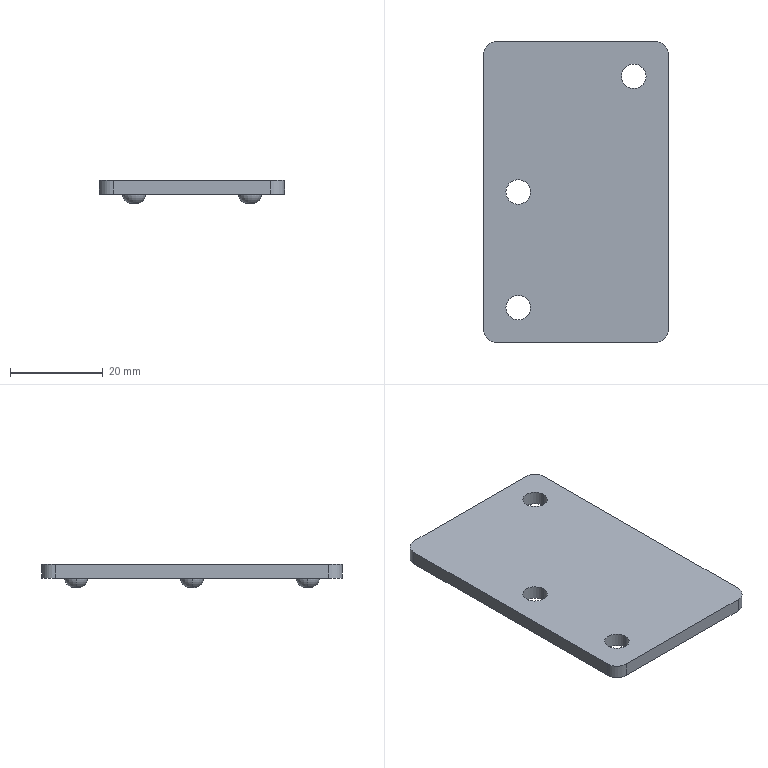Component | SolidWorks | ConnectingPlate-1 | 1 solid | 25 faces | box 40 x 65 x 5 mm | volume 7663 mm3 | cylinder 10 | plane 9 | torus 6 | commonest cylinder face diameters 5.3 x6 6 x4 | material Plain Carbon Steel
STEP:
#1=COLOUR_RGB('',0.7922,0.8196,0.9333);
#2=FILL_AREA_STYLE_COLOUR('',#1);
#3=FILL_AREA_STYLE('',(#2));
#4=SURFACE_STYLE_FILL_AREA(#3);
#5=SURFACE_SIDE_STYLE('',(#4));
#6=SURFACE_STYLE_USAGE(.BOTH.,#5);
#7=PRESENTATION_STYLE_ASSIGNMENT((#6));
#8=CARTESIAN_POINT('',(-206.949,336.302,264.226));
#9=VERTEX_POINT('',#8);
#10=CARTESIAN_POINT('',(-207.146,336.302,264.226));
#11=VERTEX_POINT('',#10);
#12=CARTESIAN_POINT('',(-207.047,336.302,264.226));
#13=DIRECTION('',(-0.,-0.,-1.));
#14=DIRECTION('',(1.,0.,-0.));
#15=AXIS2_PLACEMENT_3D('',#12,#13,#14);
#16=CIRCLE('',#15,0.09843);
#17=EDGE_CURVE('',#9,#11,#16,.T.);
#18=ORIENTED_EDGE('',*,*,#17,.T.);
#19=CARTESIAN_POINT('',(-207.067,336.302,264.147));
#20=VERTEX_POINT('',#19);
#21=CARTESIAN_POINT('',(-207.067,336.302,264.226));
#22=DIRECTION('',(0.,-1.,0.));
#23=DIRECTION('',(1.,0.,0.));
#24=AXIS2_PLACEMENT_3D('',#21,#22,#23);
#25=CIRCLE('',#24,0.07874);
#26=EDGE_CURVE('',#11,#20,#25,.T.);
#27=ORIENTED_EDGE('',*,*,#26,.T.);
#28=CARTESIAN_POINT('',(-207.028,336.302,264.147));
#29=VERTEX_POINT('',#28);
#30=CARTESIAN_POINT('',(-207.047,336.302,264.147));
#31=DIRECTION('',(-0.,-0.,-1.));
#32=DIRECTION('',(1.,0.,-0.));
#33=AXIS2_PLACEMENT_3D('',#30,#31,#32);
#34=CIRCLE('',#33,0.01969);
#35=EDGE_CURVE('',#29,#20,#34,.T.);
#36=ORIENTED_EDGE('',*,*,#35,.F.);
#37=CARTESIAN_POINT('',(-207.028,336.302,264.226));
#38=DIRECTION('',(-0.,1.,-0.));
#39=DIRECTION('',(-1.,-0.,0.));
#40=AXIS2_PLACEMENT_3D('',#37,#38,#39);
#41=CIRCLE('',#40,0.07874);
#42=EDGE_CURVE('',#9,#29,#41,.T.);
#43=ORIENTED_EDGE('',*,*,#42,.F.);
#44=EDGE_LOOP('',(#18,#27,#36,#43));
#45=FACE_OUTER_BOUND('',#44,.T.);
#46=CARTESIAN_POINT('',(-207.047,336.302,264.226));
#47=DIRECTION('',(-0.,-0.,-1.));
#48=DIRECTION('',(1.,0.,-0.));
#49=AXIS2_PLACEMENT_3D('',#46,#47,#48);
#50=TOROIDAL_SURFACE('',#49,0.01969,0.07874);
#51=ADVANCED_FACE('',(#45),#50,.T.);
#52=CARTESIAN_POINT('',(-206.949,337.286,264.226));
#53=VERTEX_POINT('',#52);
#54=CARTESIAN_POINT('',(-207.146,337.286,264.226));
#55=VERTEX_POINT('',#54);
#56=CARTESIAN_POINT('',(-207.047,337.286,264.226));
#57=DIRECTION('',(-0.,-0.,-1.));
#58=DIRECTION('',(1.,0.,-0.));
#59=AXIS2_PLACEMENT_3D('',#56,#57,#58);
#60=CIRCLE('',#59,0.09843);
#61=EDGE_CURVE('',#53,#55,#60,.T.);
#62=ORIENTED_EDGE('',*,*,#61,.T.);
#63=CARTESIAN_POINT('',(-207.067,337.286,264.147));
#64=VERTEX_POINT('',#63);
#65=CARTESIAN_POINT('',(-207.067,337.286,264.226));
#66=DIRECTION('',(0.,-1.,0.));
#67=DIRECTION('',(1.,0.,0.));
#68=AXIS2_PLACEMENT_3D('',#65,#66,#67);
#69=CIRCLE('',#68,0.07874);
#70=EDGE_CURVE('',#55,#64,#69,.T.);
#71=ORIENTED_EDGE('',*,*,#70,.T.);
#72=CARTESIAN_POINT('',(-207.028,337.286,264.147));
#73=VERTEX_POINT('',#72);
#74=CARTESIAN_POINT('',(-207.047,337.286,264.147));
#75=DIRECTION('',(-0.,-0.,-1.));
#76=DIRECTION('',(1.,0.,-0.));
#77=AXIS2_PLACEMENT_3D('',#74,#75,#76);
#78=CIRCLE('',#77,0.01969);
#79=EDGE_CURVE('',#73,#64,#78,.T.);
#80=ORIENTED_EDGE('',*,*,#79,.F.);
#81=CARTESIAN_POINT('',(-207.028,337.286,264.226));
#82=DIRECTION('',(-0.,1.,-0.));
#83=DIRECTION('',(-1.,-0.,0.));
#84=AXIS2_PLACEMENT_3D('',#81,#82,#83);
#85=CIRCLE('',#84,0.07874);
#86=EDGE_CURVE('',#53,#73,#85,.T.);
#87=ORIENTED_EDGE('',*,*,#86,.F.);
#88=EDGE_LOOP('',(#62,#71,#80,#87));
#89=FACE_OUTER_BOUND('',#88,.T.);
#90=CARTESIAN_POINT('',(-207.047,337.286,264.226));
#91=DIRECTION('',(-0.,-0.,-1.));
#92=DIRECTION('',(1.,0.,-0.));
#93=AXIS2_PLACEMENT_3D('',#90,#91,#92);
#94=TOROIDAL_SURFACE('',#93,0.01969,0.07874);
#95=ADVANCED_FACE('',(#89),#94,.T.);
#96=CARTESIAN_POINT('',(-207.933,338.27,264.226));
#97=VERTEX_POINT('',#96);
#98=CARTESIAN_POINT('',(-208.13,338.27,264.226));
#99=VERTEX_POINT('',#98);
#100=CARTESIAN_POINT('',(-208.032,338.27,264.226));
#101=DIRECTION('',(-0.,-0.,-1.));
#102=DIRECTION('',(1.,0.,-0.));
#103=AXIS2_PLACEMENT_3D('',#100,#101,#102);
#104=CIRCLE('',#103,0.09843);
#105=EDGE_CURVE('',#97,#99,#104,.T.);
#106=ORIENTED_EDGE('',*,*,#105,.T.);
#107=CARTESIAN_POINT('',(-208.051,338.27,264.147));
#108=VERTEX_POINT('',#107);
#109=CARTESIAN_POINT('',(-208.051,338.27,264.226));
#110=DIRECTION('',(0.,-1.,0.));
#111=DIRECTION('',(1.,0.,0.));
#112=AXIS2_PLACEMENT_3D('',#109,#110,#111);
#113=CIRCLE('',#112,0.07874);
#114=EDGE_CURVE('',#99,#108,#113,.T.);
#115=ORIENTED_EDGE('',*,*,#114,.T.);
#116=CARTESIAN_POINT('',(-208.012,338.27,264.147));
#117=VERTEX_POINT('',#116);
#118=CARTESIAN_POINT('',(-208.032,338.27,264.147));
#119=DIRECTION('',(-0.,-0.,-1.));
#120=DIRECTION('',(1.,0.,-0.));
#121=AXIS2_PLACEMENT_3D('',#118,#119,#120);
#122=CIRCLE('',#121,0.01969);
#123=EDGE_CURVE('',#117,#108,#122,.T.);
#124=ORIENTED_EDGE('',*,*,#123,.F.);
#125=CARTESIAN_POINT('',(-208.012,338.27,264.226));
#126=DIRECTION('',(-0.,1.,-0.));
#127=DIRECTION('',(-1.,-0.,0.));
#128=AXIS2_PLACEMENT_3D('',#125,#126,#127);
#129=CIRCLE('',#128,0.07874);
#130=EDGE_CURVE('',#97,#117,#129,.T.);
#131=ORIENTED_EDGE('',*,*,#130,.F.);
#132=EDGE_LOOP('',(#106,#115,#124,#131));
#133=FACE_OUTER_BOUND('',#132,.T.);
#134=CARTESIAN_POINT('',(-208.032,338.27,264.226));
#135=DIRECTION('',(-0.,-0.,-1.));
#136=DIRECTION('',(1.,0.,-0.));
#137=AXIS2_PLACEMENT_3D('',#134,#135,#136);
#138=TOROIDAL_SURFACE('',#137,0.01969,0.07874);
#139=ADVANCED_FACE('',(#133),#138,.T.);
#140=CARTESIAN_POINT('',(-208.136,336.302,264.226));
#141=VERTEX_POINT('',#140);
#142=CARTESIAN_POINT('',(-207.927,336.302,264.226));
#143=VERTEX_POINT('',#142);
#144=CARTESIAN_POINT('',(-208.032,336.302,264.226));
#145=DIRECTION('',(-0.,-0.,-1.));
#146=DIRECTION('',(1.,0.,-0.));
#147=AXIS2_PLACEMENT_3D('',#144,#145,#146);
#148=CIRCLE('',#147,0.1043);
#149=EDGE_CURVE('',#141,#143,#148,.T.);
#150=ORIENTED_EDGE('',*,*,#149,.T.);
#151=CARTESIAN_POINT('',(-207.927,336.302,264.344));
#152=VERTEX_POINT('',#151);
#153=CARTESIAN_POINT('',(-207.927,336.302,264.226));
#154=DIRECTION('',(0.,0.,1.));
#155=VECTOR('',#154,39.37);
#156=LINE('',#153,#155);
#157=EDGE_CURVE('',#143,#152,#156,.T.);
#158=ORIENTED_EDGE('',*,*,#157,.T.);
#159=CARTESIAN_POINT('',(-208.136,336.302,264.344));
#160=VERTEX_POINT('',#159);
#161=CARTESIAN_POINT('',(-208.032,336.302,264.344));
#162=DIRECTION('',(-0.,-0.,-1.));
#163=DIRECTION('',(1.,0.,-0.));
#164=AXIS2_PLACEMENT_3D('',#161,#162,#163);
#165=CIRCLE('',#164,0.1043);
#166=EDGE_CURVE('',#160,#152,#165,.T.);
#167=ORIENTED_EDGE('',*,*,#166,.F.);
#168=CARTESIAN_POINT('',(-208.136,336.302,264.226));
#169=DIRECTION('',(0.,0.,1.));
#170=VECTOR('',#169,39.37);
#171=LINE('',#168,#170);
#172=EDGE_CURVE('',#141,#160,#171,.T.);
#173=ORIENTED_EDGE('',*,*,#172,.F.);
#174=EDGE_LOOP('',(#150,#158,#167,#173));
#175=FACE_OUTER_BOUND('',#174,.T.);
#176=CARTESIAN_POINT('',(-208.032,336.302,264.226));
#177=DIRECTION('',(0.,0.,1.));
#178=DIRECTION('',(-1.,-0.,0.));
#179=AXIS2_PLACEMENT_3D('',#176,#177,#178);
#180=CYLINDRICAL_SURFACE('',#179,0.1043);
#181=ADVANCED_FACE('',(#175),#180,.F.);
#182=CARTESIAN_POINT('',(-207.152,338.27,264.226));
#183=VERTEX_POINT('',#182);
#184=CARTESIAN_POINT('',(-206.943,338.27,264.226));
#185=VERTEX_POINT('',#184);
#186=CARTESIAN_POINT('',(-207.047,338.27,264.226));
#187=DIRECTION('',(-0.,-0.,-1.));
#188=DIRECTION('',(1.,0.,-0.));
#189=AXIS2_PLACEMENT_3D('',#186,#187,#188);
#190=CIRCLE('',#189,0.1043);
#191=EDGE_CURVE('',#183,#185,#190,.T.);
#192=ORIENTED_EDGE('',*,*,#191,.T.);
#193=CARTESIAN_POINT('',(-206.943,338.27,264.344));
#194=VERTEX_POINT('',#193);
#195=CARTESIAN_POINT('',(-206.943,338.27,264.226));
#196=DIRECTION('',(0.,0.,1.));
#197=VECTOR('',#196,39.37);
#198=LINE('',#195,#197);
#199=EDGE_CURVE('',#185,#194,#198,.T.);
#200=ORIENTED_EDGE('',*,*,#199,.T.);
#201=CARTESIAN_POINT('',(-207.152,338.27,264.344));
#202=VERTEX_POINT('',#201);
#203=CARTESIAN_POINT('',(-207.047,338.27,264.344));
#204=DIRECTION('',(-0.,-0.,-1.));
#205=DIRECTION('',(1.,0.,-0.));
#206=AXIS2_PLACEMENT_3D('',#203,#204,#205);
#207=CIRCLE('',#206,0.1043);
#208=EDGE_CURVE('',#202,#194,#207,.T.);
#209=ORIENTED_EDGE('',*,*,#208,.F.);
#210=CARTESIAN_POINT('',(-207.152,338.27,264.226));
#211=DIRECTION('',(0.,0.,1.));
#212=VECTOR('',#211,39.37);
#213=LINE('',#210,#212);
#214=EDGE_CURVE('',#183,#202,#213,.T.);
#215=ORIENTED_EDGE('',*,*,#214,.F.);
#216=EDGE_LOOP('',(#192,#200,#209,#215));
#217=FACE_OUTER_BOUND('',#216,.T.);
#218=CARTESIAN_POINT('',(-207.047,338.27,264.226));
#219=DIRECTION('',(0.,0.,1.));
#220=DIRECTION('',(-1.,-0.,0.));
#221=AXIS2_PLACEMENT_3D('',#218,#219,#220);
#222=CYLINDRICAL_SURFACE('',#221,0.1043);
#223=ADVANCED_FACE('',(#217),#222,.F.);
#224=CARTESIAN_POINT('',(-208.136,337.286,264.226));
#225=VERTEX_POINT('',#224);
#226=CARTESIAN_POINT('',(-207.927,337.286,264.226));
#227=VERTEX_POINT('',#226);
#228=CARTESIAN_POINT('',(-208.032,337.286,264.226));
#229=DIRECTION('',(-0.,-0.,-1.));
#230=DIRECTION('',(1.,0.,-0.));
#231=AXIS2_PLACEMENT_3D('',#228,#229,#230);
#232=CIRCLE('',#231,0.1043);
#233=EDGE_CURVE('',#225,#227,#232,.T.);
#234=ORIENTED_EDGE('',*,*,#233,.T.);
#235=CARTESIAN_POINT('',(-207.927,337.286,264.344));
#236=VERTEX_POINT('',#235);
#237=CARTESIAN_POINT('',(-207.927,337.286,264.226));
#238=DIRECTION('',(0.,0.,1.));
#239=VECTOR('',#238,39.37);
#240=LINE('',#237,#239);
#241=EDGE_CURVE('',#227,#236,#240,.T.);
#242=ORIENTED_EDGE('',*,*,#241,.T.);
#243=CARTESIAN_POINT('',(-208.136,337.286,264.344));
#244=VERTEX_POINT('',#243);
#245=CARTESIAN_POINT('',(-208.032,337.286,264.344));
#246=DIRECTION('',(-0.,-0.,-1.));
#247=DIRECTION('',(1.,0.,-0.));
#248=AXIS2_PLACEMENT_3D('',#245,#246,#247);
#249=CIRCLE('',#248,0.1043);
#250=EDGE_CURVE('',#244,#236,#249,.T.);
#251=ORIENTED_EDGE('',*,*,#250,.F.);
#252=CARTESIAN_POINT('',(-208.136,337.286,264.226));
#253=DIRECTION('',(0.,0.,1.));
#254=VECTOR('',#253,39.37);
#255=LINE('',#252,#254);
#256=EDGE_CURVE('',#225,#244,#255,.T.);
#257=ORIENTED_EDGE('',*,*,#256,.F.);
#258=EDGE_LOOP('',(#234,#242,#251,#257));
#259=FACE_OUTER_BOUND('',#258,.T.);
#260=CARTESIAN_POINT('',(-208.032,337.286,264.226));
#261=DIRECTION('',(0.,0.,1.));
#262=DIRECTION('',(-1.,-0.,0.));
#263=AXIS2_PLACEMENT_3D('',#260,#261,#262);
#264=CYLINDRICAL_SURFACE('',#263,0.1043);
#265=ADVANCED_FACE('',(#259),#264,.F.);
#266=ORIENTED_EDGE('',*,*,#17,.F.);
#267=CARTESIAN_POINT('',(-207.047,336.302,264.226));
#268=DIRECTION('',(-0.,-0.,-1.));
#269=DIRECTION('',(1.,0.,-0.));
#270=AXIS2_PLACEMENT_3D('',#267,#268,#269);
#271=CIRCLE('',#270,0.09843);
#272=EDGE_CURVE('',#11,#9,#271,.T.);
#273=ORIENTED_EDGE('',*,*,#272,.F.);
#274=EDGE_LOOP('',(#266,#273));
#275=FACE_BOUND('',#274,.T.);
#276=ORIENTED_EDGE('',*,*,#61,.F.);
#277=CARTESIAN_POINT('',(-207.047,337.286,264.226));
#278=DIRECTION('',(-0.,-0.,-1.));
#279=DIRECTION('',(1.,0.,-0.));
#280=AXIS2_PLACEMENT_3D('',#277,#278,#279);
#281=CIRCLE('',#280,0.09843);
#282=EDGE_CURVE('',#55,#53,#281,.T.);
#283=ORIENTED_EDGE('',*,*,#282,.F.);
#284=EDGE_LOOP('',(#276,#283));
#285=FACE_BOUND('',#284,.T.);
#286=ORIENTED_EDGE('',*,*,#105,.F.);
#287=CARTESIAN_POINT('',(-208.032,338.27,264.226));
#288=DIRECTION('',(-0.,-0.,-1.));
#289=DIRECTION('',(1.,0.,-0.));
#290=AXIS2_PLACEMENT_3D('',#287,#288,#289);
#291=CIRCLE('',#290,0.09843);
#292=EDGE_CURVE('',#99,#97,#291,.T.);
#293=ORIENTED_EDGE('',*,*,#292,.F.);
#294=EDGE_LOOP('',(#286,#293));
#295=FACE_BOUND('',#294,.T.);
#296=ORIENTED_EDGE('',*,*,#191,.F.);
#297=CARTESIAN_POINT('',(-207.047,338.27,264.226));
#298=DIRECTION('',(-0.,-0.,-1.));
#299=DIRECTION('',(1.,0.,-0.));
#300=AXIS2_PLACEMENT_3D('',#297,#298,#299);
#301=CIRCLE('',#300,0.1043);
#302=EDGE_CURVE('',#185,#183,#301,.T.);
#303=ORIENTED_EDGE('',*,*,#302,.F.);
#304=EDGE_LOOP('',(#296,#303));
#305=FACE_BOUND('',#304,.T.);
#306=CARTESIAN_POINT('',(-206.752,336.125,264.226));
#307=VERTEX_POINT('',#306);
#308=CARTESIAN_POINT('',(-206.87,336.006,264.226));
#309=VERTEX_POINT('',#308);
#310=CARTESIAN_POINT('',(-206.87,336.125,264.226));
#311=DIRECTION('',(-0.,-0.,-1.));
#312=DIRECTION('',(1.,0.,-0.));
#313=AXIS2_PLACEMENT_3D('',#310,#311,#312);
#314=CIRCLE('',#313,0.1181);
#315=EDGE_CURVE('',#307,#309,#314,.T.);
#316=ORIENTED_EDGE('',*,*,#315,.T.);
#317=CARTESIAN_POINT('',(-208.209,336.006,264.226));
#318=VERTEX_POINT('',#317);
#319=CARTESIAN_POINT('',(-208.209,336.006,264.226));
#320=DIRECTION('',(-1.,-0.,0.));
#321=VECTOR('',#320,39.37);
#322=LINE('',#319,#321);
#323=EDGE_CURVE('',#309,#318,#322,.T.);
#324=ORIENTED_EDGE('',*,*,#323,.T.);
#325=CARTESIAN_POINT('',(-208.327,336.125,264.226));
#326=VERTEX_POINT('',#325);
#327=CARTESIAN_POINT('',(-208.209,336.125,264.226));
#328=DIRECTION('',(-0.,-0.,-1.));
#329=DIRECTION('',(1.,0.,-0.));
#330=AXIS2_PLACEMENT_3D('',#327,#328,#329);
#331=CIRCLE('',#330,0.1181);
#332=EDGE_CURVE('',#318,#326,#331,.T.);
#333=ORIENTED_EDGE('',*,*,#332,.T.);
#334=CARTESIAN_POINT('',(-208.327,338.447,264.226));
#335=VERTEX_POINT('',#334);
#336=CARTESIAN_POINT('',(-208.327,338.447,264.226));
#337=DIRECTION('',(-0.,1.,-0.));
#338=VECTOR('',#337,39.37);
#339=LINE('',#336,#338);
#340=EDGE_CURVE('',#326,#335,#339,.T.);
#341=ORIENTED_EDGE('',*,*,#340,.T.);
#342=CARTESIAN_POINT('',(-208.209,338.566,264.226));
#343=VERTEX_POINT('',#342);
#344=CARTESIAN_POINT('',(-208.209,338.447,264.226));
#345=DIRECTION('',(-0.,-0.,-1.));
#346=DIRECTION('',(-1.,-0.,0.));
#347=AXIS2_PLACEMENT_3D('',#344,#345,#346);
#348=CIRCLE('',#347,0.1181);
#349=EDGE_CURVE('',#335,#343,#348,.T.);
#350=ORIENTED_EDGE('',*,*,#349,.T.);
#351=CARTESIAN_POINT('',(-206.87,338.566,264.226));
#352=VERTEX_POINT('',#351);
#353=CARTESIAN_POINT('',(-208.209,338.566,264.226));
#354=DIRECTION('',(1.,0.,-0.));
#355=VECTOR('',#354,39.37);
#356=LINE('',#353,#355);
#357=EDGE_CURVE('',#343,#352,#356,.T.);
#358=ORIENTED_EDGE('',*,*,#357,.T.);
#359=CARTESIAN_POINT('',(-206.752,338.447,264.226));
#360=VERTEX_POINT('',#359);
#361=CARTESIAN_POINT('',(-206.87,338.447,264.226));
#362=DIRECTION('',(-0.,-0.,-1.));
#363=DIRECTION('',(-1.,-0.,0.));
#364=AXIS2_PLACEMENT_3D('',#361,#362,#363);
#365=CIRCLE('',#364,0.1181);
#366=EDGE_CURVE('',#352,#360,#365,.T.);
#367=ORIENTED_EDGE('',*,*,#366,.T.);
#368=CARTESIAN_POINT('',(-206.752,338.447,264.226));
#369=DIRECTION('',(0.,-1.,0.));
#370=VECTOR('',#369,39.37);
#371=LINE('',#368,#370);
#372=EDGE_CURVE('',#360,#307,#371,.T.);
#373=ORIENTED_EDGE('',*,*,#372,.T.);
#374=EDGE_LOOP('',(#316,#324,#333,#341,#350,#358,#367,#373));
#375=FACE_OUTER_BOUND('',#374,.T.);
#376=ORIENTED_EDGE('',*,*,#233,.F.);
#377=CARTESIAN_POINT('',(-208.032,337.286,264.226));
#378=DIRECTION('',(-0.,-0.,-1.));
#379=DIRECTION('',(1.,0.,-0.));
#380=AXIS2_PLACEMENT_3D('',#377,#378,#379);
#381=CIRCLE('',#380,0.1043);
#382=EDGE_CURVE('',#227,#225,#381,.T.);
#383=ORIENTED_EDGE('',*,*,#382,.F.);
#384=EDGE_LOOP('',(#376,#383));
#385=FACE_BOUND('',#384,.T.);
#386=ORIENTED_EDGE('',*,*,#149,.F.);
#387=CARTESIAN_POINT('',(-208.032,336.302,264.226));
#388=DIRECTION('',(-0.,-0.,-1.));
#389=DIRECTION('',(1.,0.,-0.));
#390=AXIS2_PLACEMENT_3D('',#387,#388,#389);
#391=CIRCLE('',#390,0.1043);
#392=EDGE_CURVE('',#143,#141,#391,.T.);
#393=ORIENTED_EDGE('',*,*,#392,.F.);
#394=EDGE_LOOP('',(#386,#393));
#395=FACE_BOUND('',#394,.T.);
#396=CARTESIAN_POINT('',(-206.87,336.125,264.226));
#397=DIRECTION('',(-0.,-0.,-1.));
#398=DIRECTION('',(1.,0.,-0.));
#399=AXIS2_PLACEMENT_3D('',#396,#397,#398);
#400=PLANE('',#399);
#401=ADVANCED_FACE('',(#275,#285,#295,#305,#375,#385,#395),#400,.T.);
#402=ORIENTED_EDGE('',*,*,#208,.T.);
#403=CARTESIAN_POINT('',(-207.047,338.27,264.344));
#404=DIRECTION('',(-0.,-0.,-1.));
#405=DIRECTION('',(1.,0.,-0.));
#406=AXIS2_PLACEMENT_3D('',#403,#404,#405);
#407=CIRCLE('',#406,0.1043);
#408=EDGE_CURVE('',#194,#202,#407,.T.);
#409=ORIENTED_EDGE('',*,*,#408,.T.);
#410=EDGE_LOOP('',(#402,#409));
#411=FACE_BOUND('',#410,.T.);
#412=CARTESIAN_POINT('',(-206.752,336.125,264.344));
#413=VERTEX_POINT('',#412);
#414=CARTESIAN_POINT('',(-206.87,336.006,264.344));
#415=VERTEX_POINT('',#414);
#416=CARTESIAN_POINT('',(-206.87,336.125,264.344));
#417=DIRECTION('',(-0.,-0.,-1.));
#418=DIRECTION('',(1.,0.,-0.));
#419=AXIS2_PLACEMENT_3D('',#416,#417,#418);
#420=CIRCLE('',#419,0.1181);
#421=EDGE_CURVE('',#413,#415,#420,.T.);
#422=ORIENTED_EDGE('',*,*,#421,.F.);
#423=CARTESIAN_POINT('',(-206.752,338.447,264.344));
#424=VERTEX_POINT('',#423);
#425=CARTESIAN_POINT('',(-206.752,338.447,264.344));
#426=DIRECTION('',(0.,-1.,0.));
#427=VECTOR('',#426,39.37);
#428=LINE('',#425,#427);
#429=EDGE_CURVE('',#424,#413,#428,.T.);
#430=ORIENTED_EDGE('',*,*,#429,.F.);
#431=CARTESIAN_POINT('',(-206.87,338.566,264.344));
#432=VERTEX_POINT('',#431);
#433=CARTESIAN_POINT('',(-206.87,338.447,264.344));
#434=DIRECTION('',(-0.,-0.,-1.));
#435=DIRECTION('',(-1.,-0.,0.));
#436=AXIS2_PLACEMENT_3D('',#433,#434,#435);
#437=CIRCLE('',#436,0.1181);
#438=EDGE_CURVE('',#432,#424,#437,.T.);
#439=ORIENTED_EDGE('',*,*,#438,.F.);
#440=CARTESIAN_POINT('',(-208.209,338.566,264.344));
#441=VERTEX_POINT('',#440);
#442=CARTESIAN_POINT('',(-208.209,338.566,264.344));
#443=DIRECTION('',(1.,0.,-0.));
#444=VECTOR('',#443,39.37);
#445=LINE('',#442,#444);
#446=EDGE_CURVE('',#441,#432,#445,.T.);
#447=ORIENTED_EDGE('',*,*,#446,.F.);
#448=CARTESIAN_POINT('',(-208.327,338.447,264.344));
#449=VERTEX_POINT('',#448);
#450=CARTESIAN_POINT('',(-208.209,338.447,264.344));
#451=DIRECTION('',(-0.,-0.,-1.));
#452=DIRECTION('',(-1.,-0.,0.));
#453=AXIS2_PLACEMENT_3D('',#450,#451,#452);
#454=CIRCLE('',#453,0.1181);
#455=EDGE_CURVE('',#449,#441,#454,.T.);
#456=ORIENTED_EDGE('',*,*,#455,.F.);
#457=CARTESIAN_POINT('',(-208.327,336.125,264.344));
#458=VERTEX_POINT('',#457);
#459=CARTESIAN_POINT('',(-208.327,338.447,264.344));
#460=DIRECTION('',(-0.,1.,-0.));
#461=VECTOR('',#460,39.37);
#462=LINE('',#459,#461);
#463=EDGE_CURVE('',#458,#449,#462,.T.);
#464=ORIENTED_EDGE('',*,*,#463,.F.);
#465=CARTESIAN_POINT('',(-208.209,336.006,264.344));
#466=VERTEX_POINT('',#465);
#467=CARTESIAN_POINT('',(-208.209,336.125,264.344));
#468=DIRECTION('',(-0.,-0.,-1.));
#469=DIRECTION('',(1.,0.,-0.));
#470=AXIS2_PLACEMENT_3D('',#467,#468,#469);
#471=CIRCLE('',#470,0.1181);
#472=EDGE_CURVE('',#466,#458,#471,.T.);
#473=ORIENTED_EDGE('',*,*,#472,.F.);
#474=CARTESIAN_POINT('',(-208.209,336.006,264.344));
#475=DIRECTION('',(-1.,-0.,0.));
#476=VECTOR('',#475,39.37);
#477=LINE('',#474,#476);
#478=EDGE_CURVE('',#415,#466,#477,.T.);
#479=ORIENTED_EDGE('',*,*,#478,.F.);
#480=EDGE_LOOP('',(#422,#430,#439,#447,#456,#464,#473,#479));
#481=FACE_OUTER_BOUND('',#480,.T.);
#482=ORIENTED_EDGE('',*,*,#250,.T.);
#483=CARTESIAN_POINT('',(-208.032,337.286,264.344));
#484=DIRECTION('',(-0.,-0.,-1.));
#485=DIRECTION('',(1.,0.,-0.));
#486=AXIS2_PLACEMENT_3D('',#483,#484,#485);
#487=CIRCLE('',#486,0.1043);
#488=EDGE_CURVE('',#236,#244,#487,.T.);
#489=ORIENTED_EDGE('',*,*,#488,.T.);
#490=EDGE_LOOP('',(#482,#489));
#491=FACE_BOUND('',#490,.T.);
#492=ORIENTED_EDGE('',*,*,#166,.T.);
#493=CARTESIAN_POINT('',(-208.032,336.302,264.344));
#494=DIRECTION('',(-0.,-0.,-1.));
#495=DIRECTION('',(1.,0.,-0.));
#496=AXIS2_PLACEMENT_3D('',#493,#494,#495);
#497=CIRCLE('',#496,0.1043);
#498=EDGE_CURVE('',#152,#160,#497,.T.);
#499=ORIENTED_EDGE('',*,*,#498,.T.);
#500=EDGE_LOOP('',(#492,#499));
#501=FACE_BOUND('',#500,.T.);
#502=CARTESIAN_POINT('',(-206.87,336.125,264.344));
#503=DIRECTION('',(-0.,-0.,-1.));
#504=DIRECTION('',(1.,0.,-0.));
#505=AXIS2_PLACEMENT_3D('',#502,#503,#504);
#506=PLANE('',#505);
#507=ADVANCED_FACE('',(#411,#481,#491,#501),#506,.F.);
#508=ORIENTED_EDGE('',*,*,#421,.T.);
#509=CARTESIAN_POINT('',(-206.87,336.006,264.226));
#510=DIRECTION('',(0.,0.,1.));
#511=VECTOR('',#510,39.37);
#512=LINE('',#509,#511);
#513=EDGE_CURVE('',#309,#415,#512,.T.);
#514=ORIENTED_EDGE('',*,*,#513,.F.);
#515=ORIENTED_EDGE('',*,*,#315,.F.);
#516=CARTESIAN_POINT('',(-206.752,336.125,264.226));
#517=DIRECTION('',(0.,0.,1.));
#518=VECTOR('',#517,39.37);
#519=LINE('',#516,#518);
#520=EDGE_CURVE('',#307,#413,#519,.T.);
#521=ORIENTED_EDGE('',*,*,#520,.T.);
#522=EDGE_LOOP('',(#508,#514,#515,#521));
#523=FACE_OUTER_BOUND('',#522,.T.);
#524=CARTESIAN_POINT('',(-206.87,336.125,264.226));
#525=DIRECTION('',(0.,0.,1.));
#526=DIRECTION('',(-1.,-0.,0.));
#527=AXIS2_PLACEMENT_3D('',#524,#525,#526);
#528=CYLINDRICAL_SURFACE('',#527,0.1181);
#529=ADVANCED_FACE('',(#523),#528,.T.);
#530=ORIENTED_EDGE('',*,*,#478,.T.);
#531=CARTESIAN_POINT('',(-208.209,336.006,264.226));
#532=DIRECTION('',(0.,0.,1.));
#533=VECTOR('',#532,39.37);
#534=LINE('',#531,#533);
#535=EDGE_CURVE('',#318,#466,#534,.T.);
#536=ORIENTED_EDGE('',*,*,#535,.F.);
#537=ORIENTED_EDGE('',*,*,#323,.F.);
#538=ORIENTED_EDGE('',*,*,#513,.T.);
#539=EDGE_LOOP('',(#530,#536,#537,#538));
#540=FACE_OUTER_BOUND('',#539,.T.);
#541=CARTESIAN_POINT('',(-208.209,336.006,264.226));
#542=DIRECTION('',(-0.,1.,-0.));
#543=DIRECTION('',(0.,0.,1.));
#544=AXIS2_PLACEMENT_3D('',#541,#542,#543);
#545=PLANE('',#544);
#546=ADVANCED_FACE('',(#540),#545,.F.);
#547=ORIENTED_EDGE('',*,*,#472,.T.);
#548=CARTESIAN_POINT('',(-208.327,336.125,264.226));
#549=DIRECTION('',(0.,0.,1.));
#550=VECTOR('',#549,39.37);
#551=LINE('',#548,#550);
#552=EDGE_CURVE('',#326,#458,#551,.T.);
#553=ORIENTED_EDGE('',*,*,#552,.F.);
#554=ORIENTED_EDGE('',*,*,#332,.F.);
#555=ORIENTED_EDGE('',*,*,#535,.T.);
#556=EDGE_LOOP('',(#547,#553,#554,#555));
#557=FACE_OUTER_BOUND('',#556,.T.);
#558=CARTESIAN_POINT('',(-208.209,336.125,264.226));
#559=DIRECTION('',(0.,0.,1.));
#560=DIRECTION('',(-1.,-0.,0.));
#561=AXIS2_PLACEMENT_3D('',#558,#559,#560);
#562=CYLINDRICAL_SURFACE('',#561,0.1181);
#563=ADVANCED_FACE('',(#557),#562,.T.);
#564=ORIENTED_EDGE('',*,*,#463,.T.);
#565=CARTESIAN_POINT('',(-208.327,338.447,264.226));
#566=DIRECTION('',(0.,0.,1.));
#567=VECTOR('',#566,39.37);
#568=LINE('',#565,#567);
#569=EDGE_CURVE('',#335,#449,#568,.T.);
#570=ORIENTED_EDGE('',*,*,#569,.F.);
#571=ORIENTED_EDGE('',*,*,#340,.F.);
#572=ORIENTED_EDGE('',*,*,#552,.T.);
#573=EDGE_LOOP('',(#564,#570,#571,#572));
#574=FACE_OUTER_BOUND('',#573,.T.);
#575=CARTESIAN_POINT('',(-208.327,338.447,264.226));
#576=DIRECTION('',(1.,0.,-0.));
#577=DIRECTION('',(0.,0.,1.));
#578=AXIS2_PLACEMENT_3D('',#575,#576,#577);
#579=PLANE('',#578);
#580=ADVANCED_FACE('',(#574),#579,.F.);
#581=ORIENTED_EDGE('',*,*,#455,.T.);
#582=CARTESIAN_POINT('',(-208.209,338.566,264.226));
#583=DIRECTION('',(0.,0.,1.));
#584=VECTOR('',#583,39.37);
#585=LINE('',#582,#584);
#586=EDGE_CURVE('',#343,#441,#585,.T.);
#587=ORIENTED_EDGE('',*,*,#586,.F.);
#588=ORIENTED_EDGE('',*,*,#349,.F.);
#589=ORIENTED_EDGE('',*,*,#569,.T.);
#590=EDGE_LOOP('',(#581,#587,#588,#589));
#591=FACE_OUTER_BOUND('',#590,.T.);
#592=CARTESIAN_POINT('',(-208.209,338.447,264.226));
#593=DIRECTION('',(0.,0.,1.));
#594=DIRECTION('',(-1.,-0.,0.));
#595=AXIS2_PLACEMENT_3D('',#592,#593,#594);
#596=CYLINDRICAL_SURFACE('',#595,0.1181);
#597=ADVANCED_FACE('',(#591),#596,.T.);
#598=ORIENTED_EDGE('',*,*,#446,.T.);
#599=CARTESIAN_POINT('',(-206.87,338.566,264.226));
#600=DIRECTION('',(0.,0.,1.));
#601=VECTOR('',#600,39.37);
#602=LINE('',#599,#601);
#603=EDGE_CURVE('',#352,#432,#602,.T.);
#604=ORIENTED_EDGE('',*,*,#603,.F.);
#605=ORIENTED_EDGE('',*,*,#357,.F.);
#606=ORIENTED_EDGE('',*,*,#586,.T.);
#607=EDGE_LOOP('',(#598,#604,#605,#606));
#608=FACE_OUTER_BOUND('',#607,.T.);
#609=CARTESIAN_POINT('',(-208.209,338.566,264.226));
#610=DIRECTION('',(0.,-1.,0.));
#611=DIRECTION('',(-0.,-0.,-1.));
#612=AXIS2_PLACEMENT_3D('',#609,#610,#611);
#613=PLANE('',#612);
#614=ADVANCED_FACE('',(#608),#613,.F.);
#615=ORIENTED_EDGE('',*,*,#438,.T.);
#616=CARTESIAN_POINT('',(-206.752,338.447,264.226));
#617=DIRECTION('',(0.,0.,1.));
#618=VECTOR('',#617,39.37);
#619=LINE('',#616,#618);
#620=EDGE_CURVE('',#360,#424,#619,.T.);
#621=ORIENTED_EDGE('',*,*,#620,.F.);
#622=ORIENTED_EDGE('',*,*,#366,.F.);
#623=ORIENTED_EDGE('',*,*,#603,.T.);
#624=EDGE_LOOP('',(#615,#621,#622,#623));
#625=FACE_OUTER_BOUND('',#624,.T.);
#626=CARTESIAN_POINT('',(-206.87,338.447,264.226));
#627=DIRECTION('',(0.,0.,1.));
#628=DIRECTION('',(-1.,-0.,0.));
#629=AXIS2_PLACEMENT_3D('',#626,#627,#628);
#630=CYLINDRICAL_SURFACE('',#629,0.1181);
#631=ADVANCED_FACE('',(#625),#630,.T.);
#632=ORIENTED_EDGE('',*,*,#429,.T.);
#633=ORIENTED_EDGE('',*,*,#520,.F.);
#634=ORIENTED_EDGE('',*,*,#372,.F.);
#635=ORIENTED_EDGE('',*,*,#620,.T.);
#636=EDGE_LOOP('',(#632,#633,#634,#635));
#637=FACE_OUTER_BOUND('',#636,.T.);
#638=CARTESIAN_POINT('',(-206.752,338.447,264.226));
#639=DIRECTION('',(-1.,-0.,0.));
#640=DIRECTION('',(-0.,-0.,-1.));
#641=AXIS2_PLACEMENT_3D('',#638,#639,#640);
#642=PLANE('',#641);
#643=ADVANCED_FACE('',(#637),#642,.F.);
#644=ORIENTED_EDGE('',*,*,#241,.F.);
#645=ORIENTED_EDGE('',*,*,#382,.T.);
#646=ORIENTED_EDGE('',*,*,#256,.T.);
#647=ORIENTED_EDGE('',*,*,#488,.F.);
#648=EDGE_LOOP('',(#644,#645,#646,#647));
#649=FACE_OUTER_BOUND('',#648,.T.);
#650=CARTESIAN_POINT('',(-208.032,337.286,264.226));
#651=DIRECTION('',(0.,0.,1.));
#652=DIRECTION('',(-1.,-0.,0.));
#653=AXIS2_PLACEMENT_3D('',#650,#651,#652);
#654=CYLINDRICAL_SURFACE('',#653,0.1043);
#655=ADVANCED_FACE('',(#649),#654,.F.);
#656=ORIENTED_EDGE('',*,*,#199,.F.);
#657=ORIENTED_EDGE('',*,*,#302,.T.);
#658=ORIENTED_EDGE('',*,*,#214,.T.);
#659=ORIENTED_EDGE('',*,*,#408,.F.);
#660=EDGE_LOOP('',(#656,#657,#658,#659));
#661=FACE_OUTER_BOUND('',#660,.T.);
#662=CARTESIAN_POINT('',(-207.047,338.27,264.226));
#663=DIRECTION('',(0.,0.,1.));
#664=DIRECTION('',(-1.,-0.,0.));
#665=AXIS2_PLACEMENT_3D('',#662,#663,#664);
#666=CYLINDRICAL_SURFACE('',#665,0.1043);
#667=ADVANCED_FACE('',(#661),#666,.F.);
#668=ORIENTED_EDGE('',*,*,#157,.F.);
#669=ORIENTED_EDGE('',*,*,#392,.T.);
#670=ORIENTED_EDGE('',*,*,#172,.T.);
#671=ORIENTED_EDGE('',*,*,#498,.F.);
#672=EDGE_LOOP('',(#668,#669,#670,#671));
#673=FACE_OUTER_BOUND('',#672,.T.);
#674=CARTESIAN_POINT('',(-208.032,336.302,264.226));
#675=DIRECTION('',(0.,0.,1.));
#676=DIRECTION('',(-1.,-0.,0.));
#677=AXIS2_PLACEMENT_3D('',#674,#675,#676);
#678=CYLINDRICAL_SURFACE('',#677,0.1043);
#679=ADVANCED_FACE('',(#673),#678,.F.);
#680=ORIENTED_EDGE('',*,*,#123,.T.);
#681=CARTESIAN_POINT('',(-208.032,338.27,264.147));
#682=DIRECTION('',(-0.,-0.,-1.));
#683=DIRECTION('',(1.,0.,-0.));
#684=AXIS2_PLACEMENT_3D('',#681,#682,#683);
#685=CIRCLE('',#684,0.01969);
#686=EDGE_CURVE('',#108,#117,#685,.T.);
#687=ORIENTED_EDGE('',*,*,#686,.T.);
#688=EDGE_LOOP('',(#680,#687));
#689=FACE_OUTER_BOUND('',#688,.T.);
#690=CARTESIAN_POINT('',(-208.032,338.27,264.147));
#691=DIRECTION('',(-0.,-0.,-1.));
#692=DIRECTION('',(1.,0.,-0.));
#693=AXIS2_PLACEMENT_3D('',#690,#691,#692);
#694=PLANE('',#693);
#695=ADVANCED_FACE('',(#689),#694,.T.);
#696=ORIENTED_EDGE('',*,*,#79,.T.);
#697=CARTESIAN_POINT('',(-207.047,337.286,264.147));
#698=DIRECTION('',(-0.,-0.,-1.));
#699=DIRECTION('',(1.,0.,-0.));
#700=AXIS2_PLACEMENT_3D('',#697,#698,#699);
#701=CIRCLE('',#700,0.01969);
#702=EDGE_CURVE('',#64,#73,#701,.T.);
#703=ORIENTED_EDGE('',*,*,#702,.T.);
#704=EDGE_LOOP('',(#696,#703));
#705=FACE_OUTER_BOUND('',#704,.T.);
#706=CARTESIAN_POINT('',(-207.047,337.286,264.147));
#707=DIRECTION('',(-0.,-0.,-1.));
#708=DIRECTION('',(1.,0.,-0.));
#709=AXIS2_PLACEMENT_3D('',#706,#707,#708);
#710=PLANE('',#709);
#711=ADVANCED_FACE('',(#705),#710,.T.);
#712=ORIENTED_EDGE('',*,*,#35,.T.);
#713=CARTESIAN_POINT('',(-207.047,336.302,264.147));
#714=DIRECTION('',(-0.,-0.,-1.));
#715=DIRECTION('',(1.,0.,-0.));
#716=AXIS2_PLACEMENT_3D('',#713,#714,#715);
#717=CIRCLE('',#716,0.01969);
#718=EDGE_CURVE('',#20,#29,#717,.T.);
#719=ORIENTED_EDGE('',*,*,#718,.T.);
#720=EDGE_LOOP('',(#712,#719));
#721=FACE_OUTER_BOUND('',#720,.T.);
#722=CARTESIAN_POINT('',(-207.047,336.302,264.147));
#723=DIRECTION('',(-0.,-0.,-1.));
#724=DIRECTION('',(1.,0.,-0.));
#725=AXIS2_PLACEMENT_3D('',#722,#723,#724);
#726=PLANE('',#725);
#727=ADVANCED_FACE('',(#721),#726,.T.);
#728=ORIENTED_EDGE('',*,*,#114,.F.);
#729=ORIENTED_EDGE('',*,*,#292,.T.);
#730=ORIENTED_EDGE('',*,*,#130,.T.);
#731=ORIENTED_EDGE('',*,*,#686,.F.);
#732=EDGE_LOOP('',(#728,#729,#730,#731));
#733=FACE_OUTER_BOUND('',#732,.T.);
#734=CARTESIAN_POINT('',(-208.032,338.27,264.226));
#735=DIRECTION('',(-0.,-0.,-1.));
#736=DIRECTION('',(1.,0.,-0.));
#737=AXIS2_PLACEMENT_3D('',#734,#735,#736);
#738=TOROIDAL_SURFACE('',#737,0.01969,0.07874);
#739=ADVANCED_FACE('',(#733),#738,.T.);
#740=ORIENTED_EDGE('',*,*,#70,.F.);
#741=ORIENTED_EDGE('',*,*,#282,.T.);
#742=ORIENTED_EDGE('',*,*,#86,.T.);
#743=ORIENTED_EDGE('',*,*,#702,.F.);
#744=EDGE_LOOP('',(#740,#741,#742,#743));
#745=FACE_OUTER_BOUND('',#744,.T.);
#746=CARTESIAN_POINT('',(-207.047,337.286,264.226));
#747=DIRECTION('',(-0.,-0.,-1.));
#748=DIRECTION('',(1.,0.,-0.));
#749=AXIS2_PLACEMENT_3D('',#746,#747,#748);
#750=TOROIDAL_SURFACE('',#749,0.01969,0.07874);
#751=ADVANCED_FACE('',(#745),#750,.T.);
#752=ORIENTED_EDGE('',*,*,#26,.F.);
#753=ORIENTED_EDGE('',*,*,#272,.T.);
#754=ORIENTED_EDGE('',*,*,#42,.T.);
#755=ORIENTED_EDGE('',*,*,#718,.F.);
#756=EDGE_LOOP('',(#752,#753,#754,#755));
#757=FACE_OUTER_BOUND('',#756,.T.);
#758=CARTESIAN_POINT('',(-207.047,336.302,264.226));
#759=DIRECTION('',(-0.,-0.,-1.));
#760=DIRECTION('',(1.,0.,-0.));
#761=AXIS2_PLACEMENT_3D('',#758,#759,#760);
#762=TOROIDAL_SURFACE('',#761,0.01969,0.07874);
#763=ADVANCED_FACE('',(#757),#762,.T.);
#764=CLOSED_SHELL('',(#51,#95,#139,#181,#223,#265,#401,#507,#529,#546,#563,#580,#597,#614,#631,#643,#655,#667,#679,#695,#711,#727,#739,#751,#763));
#765=MANIFOLD_SOLID_BREP('',#764);
#766=STYLED_ITEM('',(#7),#765);
#767=PRESENTATION_LAYER_ASSIGNMENT('','',(#766));
#768=CARTESIAN_POINT('',(0.,0.,0.));
#769=DIRECTION('',(0.,0.,1.));
#770=DIRECTION('',(1.,0.,0.));
#771=AXIS2_PLACEMENT_3D('',#768,#769,#770);
#772=(LENGTH_UNIT()NAMED_UNIT(*)SI_UNIT($,.METRE.));
#773=LENGTH_MEASURE_WITH_UNIT(LENGTH_MEASURE(0.0254),#772);
#774=DIMENSIONAL_EXPONENTS(1.,0.,0.,0.,0.,0.,0.);
#775=(CONVERSION_BASED_UNIT('',#773)LENGTH_UNIT()NAMED_UNIT(#774));
#776=UNCERTAINTY_MEASURE_WITH_UNIT(LENGTH_MEASURE(0.00001),#775,'','');
#777=(NAMED_UNIT(*)PLANE_ANGLE_UNIT()SI_UNIT($,.RADIAN.));
#778=(NAMED_UNIT(*)SI_UNIT($,.STERADIAN.)SOLID_ANGLE_UNIT());
#779=(GEOMETRIC_REPRESENTATION_CONTEXT(3)GLOBAL_UNCERTAINTY_ASSIGNED_CONTEXT((#776))GLOBAL_UNIT_ASSIGNED_CONTEXT((#775,#777,#778))REPRESENTATION_CONTEXT('',''));
#780=ADVANCED_BREP_SHAPE_REPRESENTATION('',(#765,#771),#779);
#781=(LENGTH_UNIT()NAMED_UNIT(*)SI_UNIT($,.METRE.));
#782=LENGTH_MEASURE_WITH_UNIT(LENGTH_MEASURE(0.0254),#781);
#783=DIMENSIONAL_EXPONENTS(1.,0.,0.,0.,0.,0.,0.);
#784=(CONVERSION_BASED_UNIT('',#782)LENGTH_UNIT()NAMED_UNIT(#783));
#785=UNCERTAINTY_MEASURE_WITH_UNIT(LENGTH_MEASURE(0.00001),#784,'','');
#786=(NAMED_UNIT(*)PLANE_ANGLE_UNIT()SI_UNIT($,.RADIAN.));
#787=(NAMED_UNIT(*)SI_UNIT($,.STERADIAN.)SOLID_ANGLE_UNIT());
#788=(GEOMETRIC_REPRESENTATION_CONTEXT(3)GLOBAL_UNCERTAINTY_ASSIGNED_CONTEXT((#785))GLOBAL_UNIT_ASSIGNED_CONTEXT((#784,#786,#787))REPRESENTATION_CONTEXT('',''));
#789=MECHANICAL_DESIGN_GEOMETRIC_PRESENTATION_REPRESENTATION('',(#766),#788);